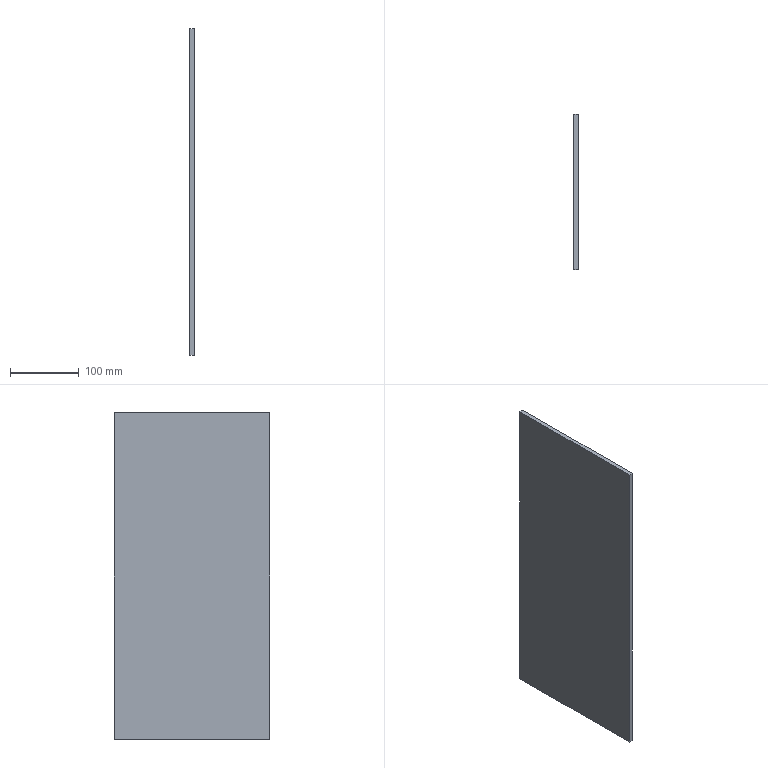Component | SolidWorks | RibPlate2-1 | 1 solid | 6 faces | box 6 x 226 x 476 mm | volume 645456 mm3 | plane 6 | material Plain Carbon Steel
STEP:
#1=COLOUR_RGB('',0.7922,0.8196,0.9333);
#2=FILL_AREA_STYLE_COLOUR('',#1);
#3=FILL_AREA_STYLE('',(#2));
#4=SURFACE_STYLE_FILL_AREA(#3);
#5=SURFACE_SIDE_STYLE('',(#4));
#6=SURFACE_STYLE_USAGE(.BOTH.,#5);
#7=PRESENTATION_STYLE_ASSIGNMENT((#6));
#8=CARTESIAN_POINT('',(31.755,53.911,65.555));
#9=VERTEX_POINT('',#8);
#10=CARTESIAN_POINT('',(31.755,53.911,84.295));
#11=VERTEX_POINT('',#10);
#12=CARTESIAN_POINT('',(31.755,53.911,65.555));
#13=DIRECTION('',(0.,-0.,1.));
#14=VECTOR('',#13,39.37);
#15=LINE('',#12,#14);
#16=EDGE_CURVE('',#9,#11,#15,.T.);
#17=ORIENTED_EDGE('',*,*,#16,.F.);
#18=CARTESIAN_POINT('',(31.519,53.911,65.555));
#19=VERTEX_POINT('',#18);
#20=CARTESIAN_POINT('',(31.519,53.911,65.555));
#21=DIRECTION('',(1.,0.,0.));
#22=VECTOR('',#21,39.37);
#23=LINE('',#20,#22);
#24=EDGE_CURVE('',#19,#9,#23,.T.);
#25=ORIENTED_EDGE('',*,*,#24,.F.);
#26=CARTESIAN_POINT('',(31.519,53.911,84.295));
#27=VERTEX_POINT('',#26);
#28=CARTESIAN_POINT('',(31.519,53.911,65.555));
#29=DIRECTION('',(0.,-0.,1.));
#30=VECTOR('',#29,39.37);
#31=LINE('',#28,#30);
#32=EDGE_CURVE('',#19,#27,#31,.T.);
#33=ORIENTED_EDGE('',*,*,#32,.T.);
#34=CARTESIAN_POINT('',(31.519,53.911,84.295));
#35=DIRECTION('',(1.,0.,0.));
#36=VECTOR('',#35,39.37);
#37=LINE('',#34,#36);
#38=EDGE_CURVE('',#27,#11,#37,.T.);
#39=ORIENTED_EDGE('',*,*,#38,.T.);
#40=EDGE_LOOP('',(#17,#25,#33,#39));
#41=FACE_OUTER_BOUND('',#40,.T.);
#42=CARTESIAN_POINT('',(31.519,53.911,65.555));
#43=DIRECTION('',(0.,1.,0.));
#44=DIRECTION('',(-1.,0.,0.));
#45=AXIS2_PLACEMENT_3D('',#42,#43,#44);
#46=PLANE('',#45);
#47=ADVANCED_FACE('',(#41),#46,.T.);
#48=CARTESIAN_POINT('',(31.755,45.014,65.555));
#49=VERTEX_POINT('',#48);
#50=CARTESIAN_POINT('',(31.755,45.014,65.555));
#51=DIRECTION('',(0.,1.,0.));
#52=VECTOR('',#51,39.37);
#53=LINE('',#50,#52);
#54=EDGE_CURVE('',#49,#9,#53,.T.);
#55=ORIENTED_EDGE('',*,*,#54,.F.);
#56=CARTESIAN_POINT('',(31.519,45.014,65.555));
#57=VERTEX_POINT('',#56);
#58=CARTESIAN_POINT('',(31.519,45.014,65.555));
#59=DIRECTION('',(1.,0.,0.));
#60=VECTOR('',#59,39.37);
#61=LINE('',#58,#60);
#62=EDGE_CURVE('',#57,#49,#61,.T.);
#63=ORIENTED_EDGE('',*,*,#62,.F.);
#64=CARTESIAN_POINT('',(31.519,45.014,65.555));
#65=DIRECTION('',(0.,1.,0.));
#66=VECTOR('',#65,39.37);
#67=LINE('',#64,#66);
#68=EDGE_CURVE('',#57,#19,#67,.T.);
#69=ORIENTED_EDGE('',*,*,#68,.T.);
#70=ORIENTED_EDGE('',*,*,#24,.T.);
#71=EDGE_LOOP('',(#55,#63,#69,#70));
#72=FACE_OUTER_BOUND('',#71,.T.);
#73=CARTESIAN_POINT('',(31.519,45.014,65.555));
#74=DIRECTION('',(0.,0.,-1.));
#75=DIRECTION('',(0.,1.,0.));
#76=AXIS2_PLACEMENT_3D('',#73,#74,#75);
#77=PLANE('',#76);
#78=ADVANCED_FACE('',(#72),#77,.T.);
#79=CARTESIAN_POINT('',(31.755,45.014,84.295));
#80=VERTEX_POINT('',#79);
#81=CARTESIAN_POINT('',(31.755,45.014,65.555));
#82=DIRECTION('',(0.,0.,-1.));
#83=VECTOR('',#82,39.37);
#84=LINE('',#81,#83);
#85=EDGE_CURVE('',#80,#49,#84,.T.);
#86=ORIENTED_EDGE('',*,*,#85,.F.);
#87=CARTESIAN_POINT('',(31.519,45.014,84.295));
#88=VERTEX_POINT('',#87);
#89=CARTESIAN_POINT('',(31.519,45.014,84.295));
#90=DIRECTION('',(1.,0.,0.));
#91=VECTOR('',#90,39.37);
#92=LINE('',#89,#91);
#93=EDGE_CURVE('',#88,#80,#92,.T.);
#94=ORIENTED_EDGE('',*,*,#93,.F.);
#95=CARTESIAN_POINT('',(31.519,45.014,65.555));
#96=DIRECTION('',(0.,0.,-1.));
#97=VECTOR('',#96,39.37);
#98=LINE('',#95,#97);
#99=EDGE_CURVE('',#88,#57,#98,.T.);
#100=ORIENTED_EDGE('',*,*,#99,.T.);
#101=ORIENTED_EDGE('',*,*,#62,.T.);
#102=EDGE_LOOP('',(#86,#94,#100,#101));
#103=FACE_OUTER_BOUND('',#102,.T.);
#104=CARTESIAN_POINT('',(31.519,45.014,65.555));
#105=DIRECTION('',(0.,-1.,-0.));
#106=DIRECTION('',(1.,0.,0.));
#107=AXIS2_PLACEMENT_3D('',#104,#105,#106);
#108=PLANE('',#107);
#109=ADVANCED_FACE('',(#103),#108,.T.);
#110=CARTESIAN_POINT('',(31.755,45.014,84.295));
#111=DIRECTION('',(0.,-1.,-0.));
#112=VECTOR('',#111,39.37);
#113=LINE('',#110,#112);
#114=EDGE_CURVE('',#11,#80,#113,.T.);
#115=ORIENTED_EDGE('',*,*,#114,.F.);
#116=ORIENTED_EDGE('',*,*,#38,.F.);
#117=CARTESIAN_POINT('',(31.519,45.014,84.295));
#118=DIRECTION('',(0.,-1.,-0.));
#119=VECTOR('',#118,39.37);
#120=LINE('',#117,#119);
#121=EDGE_CURVE('',#27,#88,#120,.T.);
#122=ORIENTED_EDGE('',*,*,#121,.T.);
#123=ORIENTED_EDGE('',*,*,#93,.T.);
#124=EDGE_LOOP('',(#115,#116,#122,#123));
#125=FACE_OUTER_BOUND('',#124,.T.);
#126=CARTESIAN_POINT('',(31.519,45.014,84.295));
#127=DIRECTION('',(0.,-0.,1.));
#128=DIRECTION('',(0.,-1.,-0.));
#129=AXIS2_PLACEMENT_3D('',#126,#127,#128);
#130=PLANE('',#129);
#131=ADVANCED_FACE('',(#125),#130,.T.);
#132=ORIENTED_EDGE('',*,*,#32,.F.);
#133=ORIENTED_EDGE('',*,*,#68,.F.);
#134=ORIENTED_EDGE('',*,*,#99,.F.);
#135=ORIENTED_EDGE('',*,*,#121,.F.);
#136=EDGE_LOOP('',(#132,#133,#134,#135));
#137=FACE_OUTER_BOUND('',#136,.T.);
#138=CARTESIAN_POINT('',(31.519,49.463,74.925));
#139=DIRECTION('',(-1.,0.,0.));
#140=DIRECTION('',(0.,-1.,-0.));
#141=AXIS2_PLACEMENT_3D('',#138,#139,#140);
#142=PLANE('',#141);
#143=ADVANCED_FACE('',(#137),#142,.T.);
#144=ORIENTED_EDGE('',*,*,#16,.T.);
#145=ORIENTED_EDGE('',*,*,#114,.T.);
#146=ORIENTED_EDGE('',*,*,#85,.T.);
#147=ORIENTED_EDGE('',*,*,#54,.T.);
#148=EDGE_LOOP('',(#144,#145,#146,#147));
#149=FACE_OUTER_BOUND('',#148,.T.);
#150=CARTESIAN_POINT('',(31.755,49.463,74.925));
#151=DIRECTION('',(-1.,0.,0.));
#152=DIRECTION('',(0.,-1.,-0.));
#153=AXIS2_PLACEMENT_3D('',#150,#151,#152);
#154=PLANE('',#153);
#155=ADVANCED_FACE('',(#149),#154,.F.);
#156=CLOSED_SHELL('',(#47,#78,#109,#131,#143,#155));
#157=MANIFOLD_SOLID_BREP('',#156);
#158=STYLED_ITEM('',(#7),#157);
#159=(LENGTH_UNIT()NAMED_UNIT(*)SI_UNIT($,.METRE.));
#160=LENGTH_MEASURE_WITH_UNIT(LENGTH_MEASURE(0.0254),#159);
#161=DIMENSIONAL_EXPONENTS(1.,0.,0.,0.,0.,0.,0.);
#162=(CONVERSION_BASED_UNIT('',#160)LENGTH_UNIT()NAMED_UNIT(#161));
#163=UNCERTAINTY_MEASURE_WITH_UNIT(LENGTH_MEASURE(0.00001),#162,'','');
#164=(NAMED_UNIT(*)PLANE_ANGLE_UNIT()SI_UNIT($,.RADIAN.));
#165=(NAMED_UNIT(*)SI_UNIT($,.STERADIAN.)SOLID_ANGLE_UNIT());
#166=(GEOMETRIC_REPRESENTATION_CONTEXT(3)GLOBAL_UNCERTAINTY_ASSIGNED_CONTEXT((#163))GLOBAL_UNIT_ASSIGNED_CONTEXT((#162,#164,#165))REPRESENTATION_CONTEXT('',''));
#167=MECHANICAL_DESIGN_GEOMETRIC_PRESENTATION_REPRESENTATION('',(#158),#166);
#168=CARTESIAN_POINT('',(0.,0.,0.));
#169=DIRECTION('',(0.,0.,1.));
#170=DIRECTION('',(1.,0.,0.));
#171=AXIS2_PLACEMENT_3D('',#168,#169,#170);
#172=(LENGTH_UNIT()NAMED_UNIT(*)SI_UNIT($,.METRE.));
#173=LENGTH_MEASURE_WITH_UNIT(LENGTH_MEASURE(0.0254),#172);
#174=DIMENSIONAL_EXPONENTS(1.,0.,0.,0.,0.,0.,0.);
#175=(CONVERSION_BASED_UNIT('',#173)LENGTH_UNIT()NAMED_UNIT(#174));
#176=UNCERTAINTY_MEASURE_WITH_UNIT(LENGTH_MEASURE(0.00001),#175,'','');
#177=(NAMED_UNIT(*)PLANE_ANGLE_UNIT()SI_UNIT($,.RADIAN.));
#178=(NAMED_UNIT(*)SI_UNIT($,.STERADIAN.)SOLID_ANGLE_UNIT());
#179=(GEOMETRIC_REPRESENTATION_CONTEXT(3)GLOBAL_UNCERTAINTY_ASSIGNED_CONTEXT((#176))GLOBAL_UNIT_ASSIGNED_CONTEXT((#175,#177,#178))REPRESENTATION_CONTEXT('',''));
#180=ADVANCED_BREP_SHAPE_REPRESENTATION('',(#157,#171),#179);
#181=PRESENTATION_LAYER_ASSIGNMENT('','',(#158));